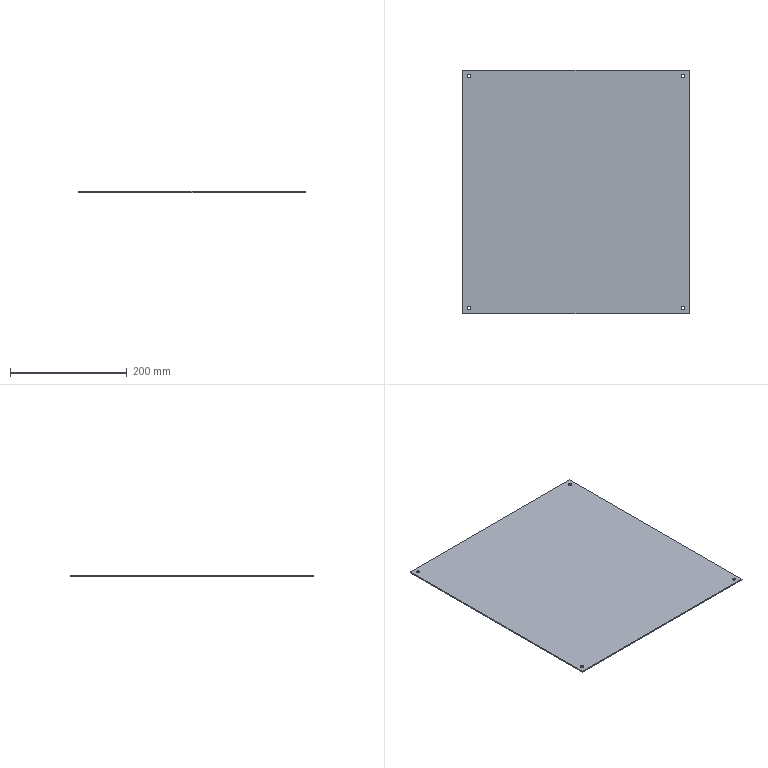Component | SolidWorks | ControlAssembly-1_ControlBoxRearPanel-1 | 1 solid | 14 faces | box 388 x 418 x 2.04 mm | volume 324142 mm3 | cylinder 8 | plane 6 | commonest cylinder face diameters 6 x8
build123d program:
from build123d import *

# Parameters (mm, degrees)
SKETCH1_W           = 388
SKETCH1_H           = 418
SKETCH1_R           = 3
BOSS_EXTRUDE1_DEPTH = 2


with BuildPart() as part:
    # Sketch1 → Boss-Extrude1 (new body)
    with BuildSketch(Plane.XY):
        with Locations((138.409, -180.814)):
            Rectangle(SKETCH1_W, SKETCH1_H)
        with Locations((-45.591, 18.186)):
            Circle(SKETCH1_R, mode=Mode.SUBTRACT)
        with Locations((322.409, 18.186)):
            Circle(SKETCH1_R, mode=Mode.SUBTRACT)
        with Locations((-45.591, -379.814)):
            Circle(SKETCH1_R, mode=Mode.SUBTRACT)
        with Locations((322.409, -379.814)):
            Circle(SKETCH1_R, mode=Mode.SUBTRACT)
    extrude(amount=BOSS_EXTRUDE1_DEPTH)


solid = part.part

# Placed as in the assembly
solid = solid.moved(Location((688.849, 425.38, 363.443), (180, -0.005652, 180)))
STEP:
#1=COLOUR_RGB('',0.7922,0.8196,0.9333);
#2=FILL_AREA_STYLE_COLOUR('',#1);
#3=FILL_AREA_STYLE('',(#2));
#4=SURFACE_STYLE_FILL_AREA(#3);
#5=SURFACE_SIDE_STYLE('',(#4));
#6=SURFACE_STYLE_USAGE(.BOTH.,#5);
#7=PRESENTATION_STYLE_ASSIGNMENT((#6));
#8=CARTESIAN_POINT('',(28.797,1.794,14.309));
#9=VERTEX_POINT('',#8);
#10=CARTESIAN_POINT('',(29.033,1.794,14.309));
#11=VERTEX_POINT('',#10);
#12=CARTESIAN_POINT('',(28.915,1.794,14.309));
#13=DIRECTION('',(0.00009864,0.,1.));
#14=DIRECTION('',(1.,0.,-0.00009864));
#15=AXIS2_PLACEMENT_3D('',#12,#13,#14);
#16=CIRCLE('',#15,0.1181);
#17=EDGE_CURVE('',#9,#11,#16,.T.);
#18=ORIENTED_EDGE('',*,*,#17,.T.);
#19=CARTESIAN_POINT('',(29.033,1.794,14.23));
#20=VERTEX_POINT('',#19);
#21=CARTESIAN_POINT('',(29.033,1.794,14.309));
#22=DIRECTION('',(-0.00009864,0.,-1.));
#23=VECTOR('',#22,39.37);
#24=LINE('',#21,#23);
#25=EDGE_CURVE('',#11,#20,#24,.T.);
#26=ORIENTED_EDGE('',*,*,#25,.T.);
#27=CARTESIAN_POINT('',(28.797,1.794,14.23));
#28=VERTEX_POINT('',#27);
#29=CARTESIAN_POINT('',(28.915,1.794,14.23));
#30=DIRECTION('',(0.00009864,0.,1.));
#31=DIRECTION('',(1.,0.,-0.00009864));
#32=AXIS2_PLACEMENT_3D('',#29,#30,#31);
#33=CIRCLE('',#32,0.1181);
#34=EDGE_CURVE('',#28,#20,#33,.T.);
#35=ORIENTED_EDGE('',*,*,#34,.F.);
#36=CARTESIAN_POINT('',(28.797,1.794,14.309));
#37=DIRECTION('',(-0.00009864,0.,-1.));
#38=VECTOR('',#37,39.37);
#39=LINE('',#36,#38);
#40=EDGE_CURVE('',#9,#28,#39,.T.);
#41=ORIENTED_EDGE('',*,*,#40,.F.);
#42=EDGE_LOOP('',(#18,#26,#35,#41));
#43=FACE_OUTER_BOUND('',#42,.T.);
#44=CARTESIAN_POINT('',(28.915,1.794,14.309));
#45=DIRECTION('',(-0.00009864,0.,-1.));
#46=DIRECTION('',(-1.,0.,0.00009864));
#47=AXIS2_PLACEMENT_3D('',#44,#45,#46);
#48=CYLINDRICAL_SURFACE('',#47,0.1181);
#49=ADVANCED_FACE('',(#43),#48,.F.);
#50=CARTESIAN_POINT('',(14.309,1.794,14.31));
#51=VERTEX_POINT('',#50);
#52=CARTESIAN_POINT('',(14.545,1.794,14.31));
#53=VERTEX_POINT('',#52);
#54=CARTESIAN_POINT('',(14.427,1.794,14.31));
#55=DIRECTION('',(0.00009864,0.,1.));
#56=DIRECTION('',(1.,0.,-0.00009864));
#57=AXIS2_PLACEMENT_3D('',#54,#55,#56);
#58=CIRCLE('',#57,0.1181);
#59=EDGE_CURVE('',#51,#53,#58,.T.);
#60=ORIENTED_EDGE('',*,*,#59,.T.);
#61=CARTESIAN_POINT('',(14.545,1.794,14.231));
#62=VERTEX_POINT('',#61);
#63=CARTESIAN_POINT('',(14.545,1.794,14.31));
#64=DIRECTION('',(-0.00009864,0.,-1.));
#65=VECTOR('',#64,39.37);
#66=LINE('',#63,#65);
#67=EDGE_CURVE('',#53,#62,#66,.T.);
#68=ORIENTED_EDGE('',*,*,#67,.T.);
#69=CARTESIAN_POINT('',(14.309,1.794,14.231));
#70=VERTEX_POINT('',#69);
#71=CARTESIAN_POINT('',(14.427,1.794,14.231));
#72=DIRECTION('',(0.00009864,0.,1.));
#73=DIRECTION('',(1.,0.,-0.00009864));
#74=AXIS2_PLACEMENT_3D('',#71,#72,#73);
#75=CIRCLE('',#74,0.1181);
#76=EDGE_CURVE('',#70,#62,#75,.T.);
#77=ORIENTED_EDGE('',*,*,#76,.F.);
#78=CARTESIAN_POINT('',(14.309,1.794,14.31));
#79=DIRECTION('',(-0.00009864,0.,-1.));
#80=VECTOR('',#79,39.37);
#81=LINE('',#78,#80);
#82=EDGE_CURVE('',#51,#70,#81,.T.);
#83=ORIENTED_EDGE('',*,*,#82,.F.);
#84=EDGE_LOOP('',(#60,#68,#77,#83));
#85=FACE_OUTER_BOUND('',#84,.T.);
#86=CARTESIAN_POINT('',(14.427,1.794,14.31));
#87=DIRECTION('',(-0.00009864,0.,-1.));
#88=DIRECTION('',(-1.,0.,0.00009864));
#89=AXIS2_PLACEMENT_3D('',#86,#87,#88);
#90=CYLINDRICAL_SURFACE('',#89,0.1181);
#91=ADVANCED_FACE('',(#85),#90,.F.);
#92=CARTESIAN_POINT('',(28.797,17.463,14.309));
#93=VERTEX_POINT('',#92);
#94=CARTESIAN_POINT('',(29.033,17.463,14.309));
#95=VERTEX_POINT('',#94);
#96=CARTESIAN_POINT('',(28.915,17.463,14.309));
#97=DIRECTION('',(0.00009864,0.,1.));
#98=DIRECTION('',(1.,0.,-0.00009864));
#99=AXIS2_PLACEMENT_3D('',#96,#97,#98);
#100=CIRCLE('',#99,0.1181);
#101=EDGE_CURVE('',#93,#95,#100,.T.);
#102=ORIENTED_EDGE('',*,*,#101,.T.);
#103=CARTESIAN_POINT('',(29.033,17.463,14.23));
#104=VERTEX_POINT('',#103);
#105=CARTESIAN_POINT('',(29.033,17.463,14.309));
#106=DIRECTION('',(-0.00009864,0.,-1.));
#107=VECTOR('',#106,39.37);
#108=LINE('',#105,#107);
#109=EDGE_CURVE('',#95,#104,#108,.T.);
#110=ORIENTED_EDGE('',*,*,#109,.T.);
#111=CARTESIAN_POINT('',(28.797,17.463,14.23));
#112=VERTEX_POINT('',#111);
#113=CARTESIAN_POINT('',(28.915,17.463,14.23));
#114=DIRECTION('',(0.00009864,0.,1.));
#115=DIRECTION('',(1.,0.,-0.00009864));
#116=AXIS2_PLACEMENT_3D('',#113,#114,#115);
#117=CIRCLE('',#116,0.1181);
#118=EDGE_CURVE('',#112,#104,#117,.T.);
#119=ORIENTED_EDGE('',*,*,#118,.F.);
#120=CARTESIAN_POINT('',(28.797,17.463,14.309));
#121=DIRECTION('',(-0.00009864,0.,-1.));
#122=VECTOR('',#121,39.37);
#123=LINE('',#120,#122);
#124=EDGE_CURVE('',#93,#112,#123,.T.);
#125=ORIENTED_EDGE('',*,*,#124,.F.);
#126=EDGE_LOOP('',(#102,#110,#119,#125));
#127=FACE_OUTER_BOUND('',#126,.T.);
#128=CARTESIAN_POINT('',(28.915,17.463,14.309));
#129=DIRECTION('',(-0.00009864,0.,-1.));
#130=DIRECTION('',(-1.,0.,0.00009864));
#131=AXIS2_PLACEMENT_3D('',#128,#129,#130);
#132=CYLINDRICAL_SURFACE('',#131,0.1181);
#133=ADVANCED_FACE('',(#127),#132,.F.);
#134=CARTESIAN_POINT('',(14.309,17.463,14.31));
#135=VERTEX_POINT('',#134);
#136=CARTESIAN_POINT('',(14.545,17.463,14.31));
#137=VERTEX_POINT('',#136);
#138=CARTESIAN_POINT('',(14.427,17.463,14.31));
#139=DIRECTION('',(0.00009864,0.,1.));
#140=DIRECTION('',(1.,0.,-0.00009864));
#141=AXIS2_PLACEMENT_3D('',#138,#139,#140);
#142=CIRCLE('',#141,0.1181);
#143=EDGE_CURVE('',#135,#137,#142,.T.);
#144=ORIENTED_EDGE('',*,*,#143,.T.);
#145=CARTESIAN_POINT('',(14.545,17.463,14.231));
#146=VERTEX_POINT('',#145);
#147=CARTESIAN_POINT('',(14.545,17.463,14.31));
#148=DIRECTION('',(-0.00009864,0.,-1.));
#149=VECTOR('',#148,39.37);
#150=LINE('',#147,#149);
#151=EDGE_CURVE('',#137,#146,#150,.T.);
#152=ORIENTED_EDGE('',*,*,#151,.T.);
#153=CARTESIAN_POINT('',(14.309,17.463,14.231));
#154=VERTEX_POINT('',#153);
#155=CARTESIAN_POINT('',(14.427,17.463,14.231));
#156=DIRECTION('',(0.00009864,0.,1.));
#157=DIRECTION('',(1.,0.,-0.00009864));
#158=AXIS2_PLACEMENT_3D('',#155,#156,#157);
#159=CIRCLE('',#158,0.1181);
#160=EDGE_CURVE('',#154,#146,#159,.T.);
#161=ORIENTED_EDGE('',*,*,#160,.F.);
#162=CARTESIAN_POINT('',(14.309,17.463,14.31));
#163=DIRECTION('',(-0.00009864,0.,-1.));
#164=VECTOR('',#163,39.37);
#165=LINE('',#162,#164);
#166=EDGE_CURVE('',#135,#154,#165,.T.);
#167=ORIENTED_EDGE('',*,*,#166,.F.);
#168=EDGE_LOOP('',(#144,#152,#161,#167));
#169=FACE_OUTER_BOUND('',#168,.T.);
#170=CARTESIAN_POINT('',(14.427,17.463,14.31));
#171=DIRECTION('',(-0.00009864,0.,-1.));
#172=DIRECTION('',(-1.,0.,0.00009864));
#173=AXIS2_PLACEMENT_3D('',#170,#171,#172);
#174=CYLINDRICAL_SURFACE('',#173,0.1181);
#175=ADVANCED_FACE('',(#169),#174,.F.);
#176=ORIENTED_EDGE('',*,*,#59,.F.);
#177=CARTESIAN_POINT('',(14.427,1.794,14.31));
#178=DIRECTION('',(0.00009864,0.,1.));
#179=DIRECTION('',(1.,0.,-0.00009864));
#180=AXIS2_PLACEMENT_3D('',#177,#178,#179);
#181=CIRCLE('',#180,0.1181);
#182=EDGE_CURVE('',#53,#51,#181,.T.);
#183=ORIENTED_EDGE('',*,*,#182,.F.);
#184=EDGE_LOOP('',(#176,#183));
#185=FACE_BOUND('',#184,.T.);
#186=ORIENTED_EDGE('',*,*,#143,.F.);
#187=CARTESIAN_POINT('',(14.427,17.463,14.31));
#188=DIRECTION('',(0.00009864,0.,1.));
#189=DIRECTION('',(1.,0.,-0.00009864));
#190=AXIS2_PLACEMENT_3D('',#187,#188,#189);
#191=CIRCLE('',#190,0.1181);
#192=EDGE_CURVE('',#137,#135,#191,.T.);
#193=ORIENTED_EDGE('',*,*,#192,.F.);
#194=EDGE_LOOP('',(#186,#193));
#195=FACE_BOUND('',#194,.T.);
#196=CARTESIAN_POINT('',(14.033,17.857,14.31));
#197=VERTEX_POINT('',#196);
#198=CARTESIAN_POINT('',(14.033,1.4,14.31));
#199=VERTEX_POINT('',#198);
#200=CARTESIAN_POINT('',(14.033,17.857,14.31));
#201=DIRECTION('',(0.,-1.,-0.));
#202=VECTOR('',#201,39.37);
#203=LINE('',#200,#202);
#204=EDGE_CURVE('',#197,#199,#203,.T.);
#205=ORIENTED_EDGE('',*,*,#204,.T.);
#206=CARTESIAN_POINT('',(29.309,1.4,14.309));
#207=VERTEX_POINT('',#206);
#208=CARTESIAN_POINT('',(14.033,1.4,14.31));
#209=DIRECTION('',(1.,0.,-0.00009864));
#210=VECTOR('',#209,39.37);
#211=LINE('',#208,#210);
#212=EDGE_CURVE('',#199,#207,#211,.T.);
#213=ORIENTED_EDGE('',*,*,#212,.T.);
#214=CARTESIAN_POINT('',(29.309,17.857,14.309));
#215=VERTEX_POINT('',#214);
#216=CARTESIAN_POINT('',(29.309,17.857,14.309));
#217=DIRECTION('',(-0.,1.,0.));
#218=VECTOR('',#217,39.37);
#219=LINE('',#216,#218);
#220=EDGE_CURVE('',#207,#215,#219,.T.);
#221=ORIENTED_EDGE('',*,*,#220,.T.);
#222=CARTESIAN_POINT('',(14.033,17.857,14.31));
#223=DIRECTION('',(-1.,0.,0.00009864));
#224=VECTOR('',#223,39.37);
#225=LINE('',#222,#224);
#226=EDGE_CURVE('',#215,#197,#225,.T.);
#227=ORIENTED_EDGE('',*,*,#226,.T.);
#228=EDGE_LOOP('',(#205,#213,#221,#227));
#229=FACE_OUTER_BOUND('',#228,.T.);
#230=ORIENTED_EDGE('',*,*,#101,.F.);
#231=CARTESIAN_POINT('',(28.915,17.463,14.309));
#232=DIRECTION('',(0.00009864,0.,1.));
#233=DIRECTION('',(1.,0.,-0.00009864));
#234=AXIS2_PLACEMENT_3D('',#231,#232,#233);
#235=CIRCLE('',#234,0.1181);
#236=EDGE_CURVE('',#95,#93,#235,.T.);
#237=ORIENTED_EDGE('',*,*,#236,.F.);
#238=EDGE_LOOP('',(#230,#237));
#239=FACE_BOUND('',#238,.T.);
#240=ORIENTED_EDGE('',*,*,#17,.F.);
#241=CARTESIAN_POINT('',(28.915,1.794,14.309));
#242=DIRECTION('',(0.00009864,0.,1.));
#243=DIRECTION('',(1.,0.,-0.00009864));
#244=AXIS2_PLACEMENT_3D('',#241,#242,#243);
#245=CIRCLE('',#244,0.1181);
#246=EDGE_CURVE('',#11,#9,#245,.T.);
#247=ORIENTED_EDGE('',*,*,#246,.F.);
#248=EDGE_LOOP('',(#240,#247));
#249=FACE_BOUND('',#248,.T.);
#250=CARTESIAN_POINT('',(16.222,16.747,14.31));
#251=DIRECTION('',(0.00009864,0.,1.));
#252=DIRECTION('',(1.,0.,-0.00009864));
#253=AXIS2_PLACEMENT_3D('',#250,#251,#252);
#254=PLANE('',#253);
#255=ADVANCED_FACE('',(#185,#195,#229,#239,#249),#254,.T.);
#256=CARTESIAN_POINT('',(14.033,17.857,14.231));
#257=VERTEX_POINT('',#256);
#258=CARTESIAN_POINT('',(14.033,1.4,14.231));
#259=VERTEX_POINT('',#258);
#260=CARTESIAN_POINT('',(14.033,17.857,14.231));
#261=DIRECTION('',(0.,-1.,-0.));
#262=VECTOR('',#261,39.37);
#263=LINE('',#260,#262);
#264=EDGE_CURVE('',#257,#259,#263,.T.);
#265=ORIENTED_EDGE('',*,*,#264,.F.);
#266=CARTESIAN_POINT('',(29.309,17.857,14.23));
#267=VERTEX_POINT('',#266);
#268=CARTESIAN_POINT('',(14.033,17.857,14.231));
#269=DIRECTION('',(-1.,0.,0.00009864));
#270=VECTOR('',#269,39.37);
#271=LINE('',#268,#270);
#272=EDGE_CURVE('',#267,#257,#271,.T.);
#273=ORIENTED_EDGE('',*,*,#272,.F.);
#274=CARTESIAN_POINT('',(29.309,1.4,14.23));
#275=VERTEX_POINT('',#274);
#276=CARTESIAN_POINT('',(29.309,17.857,14.23));
#277=DIRECTION('',(-0.,1.,0.));
#278=VECTOR('',#277,39.37);
#279=LINE('',#276,#278);
#280=EDGE_CURVE('',#275,#267,#279,.T.);
#281=ORIENTED_EDGE('',*,*,#280,.F.);
#282=CARTESIAN_POINT('',(14.033,1.4,14.231));
#283=DIRECTION('',(1.,0.,-0.00009864));
#284=VECTOR('',#283,39.37);
#285=LINE('',#282,#284);
#286=EDGE_CURVE('',#259,#275,#285,.T.);
#287=ORIENTED_EDGE('',*,*,#286,.F.);
#288=EDGE_LOOP('',(#265,#273,#281,#287));
#289=FACE_OUTER_BOUND('',#288,.T.);
#290=ORIENTED_EDGE('',*,*,#160,.T.);
#291=CARTESIAN_POINT('',(14.427,17.463,14.231));
#292=DIRECTION('',(0.00009864,0.,1.));
#293=DIRECTION('',(1.,0.,-0.00009864));
#294=AXIS2_PLACEMENT_3D('',#291,#292,#293);
#295=CIRCLE('',#294,0.1181);
#296=EDGE_CURVE('',#146,#154,#295,.T.);
#297=ORIENTED_EDGE('',*,*,#296,.T.);
#298=EDGE_LOOP('',(#290,#297));
#299=FACE_BOUND('',#298,.T.);
#300=ORIENTED_EDGE('',*,*,#118,.T.);
#301=CARTESIAN_POINT('',(28.915,17.463,14.23));
#302=DIRECTION('',(0.00009864,0.,1.));
#303=DIRECTION('',(1.,0.,-0.00009864));
#304=AXIS2_PLACEMENT_3D('',#301,#302,#303);
#305=CIRCLE('',#304,0.1181);
#306=EDGE_CURVE('',#104,#112,#305,.T.);
#307=ORIENTED_EDGE('',*,*,#306,.T.);
#308=EDGE_LOOP('',(#300,#307));
#309=FACE_BOUND('',#308,.T.);
#310=ORIENTED_EDGE('',*,*,#76,.T.);
#311=CARTESIAN_POINT('',(14.427,1.794,14.231));
#312=DIRECTION('',(0.00009864,0.,1.));
#313=DIRECTION('',(1.,0.,-0.00009864));
#314=AXIS2_PLACEMENT_3D('',#311,#312,#313);
#315=CIRCLE('',#314,0.1181);
#316=EDGE_CURVE('',#62,#70,#315,.T.);
#317=ORIENTED_EDGE('',*,*,#316,.T.);
#318=EDGE_LOOP('',(#310,#317));
#319=FACE_BOUND('',#318,.T.);
#320=ORIENTED_EDGE('',*,*,#34,.T.);
#321=CARTESIAN_POINT('',(28.915,1.794,14.23));
#322=DIRECTION('',(0.00009864,0.,1.));
#323=DIRECTION('',(1.,0.,-0.00009864));
#324=AXIS2_PLACEMENT_3D('',#321,#322,#323);
#325=CIRCLE('',#324,0.1181);
#326=EDGE_CURVE('',#20,#28,#325,.T.);
#327=ORIENTED_EDGE('',*,*,#326,.T.);
#328=EDGE_LOOP('',(#320,#327));
#329=FACE_BOUND('',#328,.T.);
#330=CARTESIAN_POINT('',(16.222,16.747,14.231));
#331=DIRECTION('',(0.00009864,0.,1.));
#332=DIRECTION('',(1.,0.,-0.00009864));
#333=AXIS2_PLACEMENT_3D('',#330,#331,#332);
#334=PLANE('',#333);
#335=ADVANCED_FACE('',(#289,#299,#309,#319,#329),#334,.F.);
#336=ORIENTED_EDGE('',*,*,#264,.T.);
#337=CARTESIAN_POINT('',(14.033,1.4,14.31));
#338=DIRECTION('',(-0.00009864,0.,-1.));
#339=VECTOR('',#338,39.37);
#340=LINE('',#337,#339);
#341=EDGE_CURVE('',#199,#259,#340,.T.);
#342=ORIENTED_EDGE('',*,*,#341,.F.);
#343=ORIENTED_EDGE('',*,*,#204,.F.);
#344=CARTESIAN_POINT('',(14.033,17.857,14.31));
#345=DIRECTION('',(-0.00009864,0.,-1.));
#346=VECTOR('',#345,39.37);
#347=LINE('',#344,#346);
#348=EDGE_CURVE('',#197,#257,#347,.T.);
#349=ORIENTED_EDGE('',*,*,#348,.T.);
#350=EDGE_LOOP('',(#336,#342,#343,#349));
#351=FACE_OUTER_BOUND('',#350,.T.);
#352=CARTESIAN_POINT('',(14.033,17.857,14.31));
#353=DIRECTION('',(1.,0.,-0.00009864));
#354=DIRECTION('',(-0.,1.,0.));
#355=AXIS2_PLACEMENT_3D('',#352,#353,#354);
#356=PLANE('',#355);
#357=ADVANCED_FACE('',(#351),#356,.F.);
#358=ORIENTED_EDGE('',*,*,#286,.T.);
#359=CARTESIAN_POINT('',(29.309,1.4,14.309));
#360=DIRECTION('',(-0.00009864,0.,-1.));
#361=VECTOR('',#360,39.37);
#362=LINE('',#359,#361);
#363=EDGE_CURVE('',#207,#275,#362,.T.);
#364=ORIENTED_EDGE('',*,*,#363,.F.);
#365=ORIENTED_EDGE('',*,*,#212,.F.);
#366=ORIENTED_EDGE('',*,*,#341,.T.);
#367=EDGE_LOOP('',(#358,#364,#365,#366));
#368=FACE_OUTER_BOUND('',#367,.T.);
#369=CARTESIAN_POINT('',(14.033,1.4,14.31));
#370=DIRECTION('',(0.,1.,0.));
#371=DIRECTION('',(0.00009864,0.,1.));
#372=AXIS2_PLACEMENT_3D('',#369,#370,#371);
#373=PLANE('',#372);
#374=ADVANCED_FACE('',(#368),#373,.F.);
#375=ORIENTED_EDGE('',*,*,#280,.T.);
#376=CARTESIAN_POINT('',(29.309,17.857,14.309));
#377=DIRECTION('',(-0.00009864,0.,-1.));
#378=VECTOR('',#377,39.37);
#379=LINE('',#376,#378);
#380=EDGE_CURVE('',#215,#267,#379,.T.);
#381=ORIENTED_EDGE('',*,*,#380,.F.);
#382=ORIENTED_EDGE('',*,*,#220,.F.);
#383=ORIENTED_EDGE('',*,*,#363,.T.);
#384=EDGE_LOOP('',(#375,#381,#382,#383));
#385=FACE_OUTER_BOUND('',#384,.T.);
#386=CARTESIAN_POINT('',(29.309,17.857,14.309));
#387=DIRECTION('',(-1.,-0.,0.00009864));
#388=DIRECTION('',(0.,-1.,-0.));
#389=AXIS2_PLACEMENT_3D('',#386,#387,#388);
#390=PLANE('',#389);
#391=ADVANCED_FACE('',(#385),#390,.F.);
#392=ORIENTED_EDGE('',*,*,#272,.T.);
#393=ORIENTED_EDGE('',*,*,#348,.F.);
#394=ORIENTED_EDGE('',*,*,#226,.F.);
#395=ORIENTED_EDGE('',*,*,#380,.T.);
#396=EDGE_LOOP('',(#392,#393,#394,#395));
#397=FACE_OUTER_BOUND('',#396,.T.);
#398=CARTESIAN_POINT('',(14.033,17.857,14.31));
#399=DIRECTION('',(0.,-1.,0.));
#400=DIRECTION('',(-0.00009864,0.,-1.));
#401=AXIS2_PLACEMENT_3D('',#398,#399,#400);
#402=PLANE('',#401);
#403=ADVANCED_FACE('',(#397),#402,.F.);
#404=ORIENTED_EDGE('',*,*,#151,.F.);
#405=ORIENTED_EDGE('',*,*,#192,.T.);
#406=ORIENTED_EDGE('',*,*,#166,.T.);
#407=ORIENTED_EDGE('',*,*,#296,.F.);
#408=EDGE_LOOP('',(#404,#405,#406,#407));
#409=FACE_OUTER_BOUND('',#408,.T.);
#410=CARTESIAN_POINT('',(14.427,17.463,14.31));
#411=DIRECTION('',(-0.00009864,0.,-1.));
#412=DIRECTION('',(-1.,0.,0.00009864));
#413=AXIS2_PLACEMENT_3D('',#410,#411,#412);
#414=CYLINDRICAL_SURFACE('',#413,0.1181);
#415=ADVANCED_FACE('',(#409),#414,.F.);
#416=ORIENTED_EDGE('',*,*,#109,.F.);
#417=ORIENTED_EDGE('',*,*,#236,.T.);
#418=ORIENTED_EDGE('',*,*,#124,.T.);
#419=ORIENTED_EDGE('',*,*,#306,.F.);
#420=EDGE_LOOP('',(#416,#417,#418,#419));
#421=FACE_OUTER_BOUND('',#420,.T.);
#422=CARTESIAN_POINT('',(28.915,17.463,14.309));
#423=DIRECTION('',(-0.00009864,0.,-1.));
#424=DIRECTION('',(-1.,0.,0.00009864));
#425=AXIS2_PLACEMENT_3D('',#422,#423,#424);
#426=CYLINDRICAL_SURFACE('',#425,0.1181);
#427=ADVANCED_FACE('',(#421),#426,.F.);
#428=ORIENTED_EDGE('',*,*,#67,.F.);
#429=ORIENTED_EDGE('',*,*,#182,.T.);
#430=ORIENTED_EDGE('',*,*,#82,.T.);
#431=ORIENTED_EDGE('',*,*,#316,.F.);
#432=EDGE_LOOP('',(#428,#429,#430,#431));
#433=FACE_OUTER_BOUND('',#432,.T.);
#434=CARTESIAN_POINT('',(14.427,1.794,14.31));
#435=DIRECTION('',(-0.00009864,0.,-1.));
#436=DIRECTION('',(-1.,0.,0.00009864));
#437=AXIS2_PLACEMENT_3D('',#434,#435,#436);
#438=CYLINDRICAL_SURFACE('',#437,0.1181);
#439=ADVANCED_FACE('',(#433),#438,.F.);
#440=ORIENTED_EDGE('',*,*,#25,.F.);
#441=ORIENTED_EDGE('',*,*,#246,.T.);
#442=ORIENTED_EDGE('',*,*,#40,.T.);
#443=ORIENTED_EDGE('',*,*,#326,.F.);
#444=EDGE_LOOP('',(#440,#441,#442,#443));
#445=FACE_OUTER_BOUND('',#444,.T.);
#446=CARTESIAN_POINT('',(28.915,1.794,14.309));
#447=DIRECTION('',(-0.00009864,0.,-1.));
#448=DIRECTION('',(-1.,0.,0.00009864));
#449=AXIS2_PLACEMENT_3D('',#446,#447,#448);
#450=CYLINDRICAL_SURFACE('',#449,0.1181);
#451=ADVANCED_FACE('',(#445),#450,.F.);
#452=CLOSED_SHELL('',(#49,#91,#133,#175,#255,#335,#357,#374,#391,#403,#415,#427,#439,#451));
#453=MANIFOLD_SOLID_BREP('',#452);
#454=STYLED_ITEM('',(#7),#453);
#455=(LENGTH_UNIT()NAMED_UNIT(*)SI_UNIT($,.METRE.));
#456=LENGTH_MEASURE_WITH_UNIT(LENGTH_MEASURE(0.0254),#455);
#457=DIMENSIONAL_EXPONENTS(1.,0.,0.,0.,0.,0.,0.);
#458=(CONVERSION_BASED_UNIT('',#456)LENGTH_UNIT()NAMED_UNIT(#457));
#459=UNCERTAINTY_MEASURE_WITH_UNIT(LENGTH_MEASURE(0.00001),#458,'','');
#460=(NAMED_UNIT(*)PLANE_ANGLE_UNIT()SI_UNIT($,.RADIAN.));
#461=(NAMED_UNIT(*)SI_UNIT($,.STERADIAN.)SOLID_ANGLE_UNIT());
#462=(GEOMETRIC_REPRESENTATION_CONTEXT(3)GLOBAL_UNCERTAINTY_ASSIGNED_CONTEXT((#459))GLOBAL_UNIT_ASSIGNED_CONTEXT((#458,#460,#461))REPRESENTATION_CONTEXT('',''));
#463=MECHANICAL_DESIGN_GEOMETRIC_PRESENTATION_REPRESENTATION('',(#454),#462);
#464=CARTESIAN_POINT('',(0.,0.,0.));
#465=DIRECTION('',(0.,0.,1.));
#466=DIRECTION('',(1.,0.,0.));
#467=AXIS2_PLACEMENT_3D('',#464,#465,#466);
#468=(LENGTH_UNIT()NAMED_UNIT(*)SI_UNIT($,.METRE.));
#469=LENGTH_MEASURE_WITH_UNIT(LENGTH_MEASURE(0.0254),#468);
#470=DIMENSIONAL_EXPONENTS(1.,0.,0.,0.,0.,0.,0.);
#471=(CONVERSION_BASED_UNIT('',#469)LENGTH_UNIT()NAMED_UNIT(#470));
#472=UNCERTAINTY_MEASURE_WITH_UNIT(LENGTH_MEASURE(0.00001),#471,'','');
#473=(NAMED_UNIT(*)PLANE_ANGLE_UNIT()SI_UNIT($,.RADIAN.));
#474=(NAMED_UNIT(*)SI_UNIT($,.STERADIAN.)SOLID_ANGLE_UNIT());
#475=(GEOMETRIC_REPRESENTATION_CONTEXT(3)GLOBAL_UNCERTAINTY_ASSIGNED_CONTEXT((#472))GLOBAL_UNIT_ASSIGNED_CONTEXT((#471,#473,#474))REPRESENTATION_CONTEXT('',''));
#476=ADVANCED_BREP_SHAPE_REPRESENTATION('',(#453,#467),#475);
#477=PRESENTATION_LAYER_ASSIGNMENT('','',(#454));